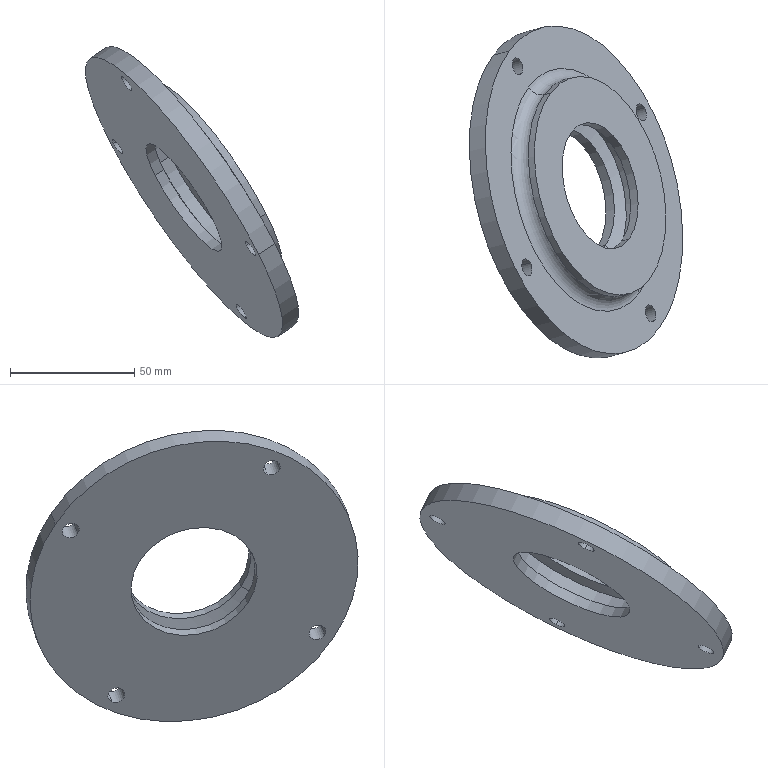Component | SolidWorks | InnerDustCover-1 | 1 solid | 27 faces | box 85.86 x 133.68 x 117.19 mm | volume 124699 mm3 | cylinder 18 | cone 4 | plane 3 | torus 2 | commonest cylinder face diameters 7 x8 52 x4 64 x2 90 x2 135 x2
STEP:
#1=CARTESIAN_POINT('',(-14.667,-7.905,-14.02));
#2=VERTEX_POINT('',#1);
#3=CARTESIAN_POINT('',(-16.423,-4.646,-12.677));
#4=VERTEX_POINT('',#3);
#5=CARTESIAN_POINT('',(-15.545,-6.275,-13.349));
#6=DIRECTION('',(-0.8088,-0.2094,-0.5495));
#7=DIRECTION('',(-0.4459,0.8276,0.341));
#8=AXIS2_PLACEMENT_3D('',#5,#6,#7);
#9=CIRCLE('',#8,1.969);
#10=EDGE_CURVE('',#2,#4,#9,.T.);
#11=ORIENTED_EDGE('',*,*,#10,.F.);
#12=CARTESIAN_POINT('',(-14.596,-7.7,-13.844));
#13=VERTEX_POINT('',#12);
#14=CARTESIAN_POINT('',(-14.508,-7.863,-13.912));
#15=DIRECTION('',(0.3834,0.5208,-0.7628));
#16=DIRECTION('',(0.,0.8259,0.5639));
#17=AXIS2_PLACEMENT_3D('',#14,#15,#16);
#18=CIRCLE('',#17,0.1969);
#19=EDGE_CURVE('',#2,#13,#18,.T.);
#20=ORIENTED_EDGE('',*,*,#19,.T.);
#21=CARTESIAN_POINT('',(-16.176,-4.768,-12.636));
#22=VERTEX_POINT('',#21);
#23=CARTESIAN_POINT('',(-15.386,-6.234,-13.24));
#24=DIRECTION('',(0.8088,0.2094,0.5495));
#25=DIRECTION('',(-0.4459,0.8276,0.341));
#26=AXIS2_PLACEMENT_3D('',#23,#24,#25);
#27=CIRCLE('',#26,1.772);
#28=EDGE_CURVE('',#22,#13,#27,.T.);
#29=ORIENTED_EDGE('',*,*,#28,.F.);
#30=CARTESIAN_POINT('',(-16.263,-4.605,-12.569));
#31=DIRECTION('',(-0.3834,-0.5208,0.7628));
#32=DIRECTION('',(0.,-0.8259,-0.5639));
#33=AXIS2_PLACEMENT_3D('',#30,#31,#32);
#34=CIRCLE('',#33,0.1969);
#35=EDGE_CURVE('',#4,#22,#34,.T.);
#36=ORIENTED_EDGE('',*,*,#35,.F.);
#37=EDGE_LOOP('',(#11,#20,#29,#36));
#38=FACE_OUTER_BOUND('',#37,.T.);
#39=CARTESIAN_POINT('',(-15.386,-6.234,-13.24));
#40=DIRECTION('',(-0.8088,-0.2094,-0.5495));
#41=DIRECTION('',(-0.4459,0.8276,0.341));
#42=AXIS2_PLACEMENT_3D('',#39,#40,#41);
#43=TOROIDAL_SURFACE('',#42,1.969,0.1969);
#44=ADVANCED_FACE('',(#38),#43,.F.);
#45=CARTESIAN_POINT('',(-14.841,-5.039,-15.429));
#46=VERTEX_POINT('',#45);
#47=CARTESIAN_POINT('',(-14.947,-5.183,-15.218));
#48=VERTEX_POINT('',#47);
#49=CARTESIAN_POINT('',(-14.894,-5.111,-15.323));
#50=DIRECTION('',(0.8088,0.2094,0.5495));
#51=DIRECTION('',(-0.3834,-0.5208,0.7628));
#52=AXIS2_PLACEMENT_3D('',#49,#50,#51);
#53=CIRCLE('',#52,0.1378);
#54=EDGE_CURVE('',#46,#48,#53,.T.);
#55=ORIENTED_EDGE('',*,*,#54,.F.);
#56=CARTESIAN_POINT('',(-14.587,-4.973,-15.255));
#57=VERTEX_POINT('',#56);
#58=CARTESIAN_POINT('',(-15.287,-5.155,-15.731));
#59=DIRECTION('',(0.8088,0.2094,0.5495));
#60=VECTOR('',#59,39.37);
#61=LINE('',#58,#60);
#62=EDGE_CURVE('',#46,#57,#61,.T.);
#63=ORIENTED_EDGE('',*,*,#62,.T.);
#64=CARTESIAN_POINT('',(-14.692,-5.117,-15.045));
#65=VERTEX_POINT('',#64);
#66=CARTESIAN_POINT('',(-14.639,-5.045,-15.15));
#67=DIRECTION('',(-0.8088,-0.2094,-0.5495));
#68=DIRECTION('',(0.3834,0.5208,-0.7628));
#69=AXIS2_PLACEMENT_3D('',#66,#67,#68);
#70=CIRCLE('',#69,0.1378);
#71=EDGE_CURVE('',#65,#57,#70,.T.);
#72=ORIENTED_EDGE('',*,*,#71,.F.);
#73=CARTESIAN_POINT('',(-15.393,-5.298,-15.521));
#74=DIRECTION('',(0.8088,0.2094,0.5495));
#75=VECTOR('',#74,39.37);
#76=LINE('',#73,#75);
#77=EDGE_CURVE('',#48,#65,#76,.T.);
#78=ORIENTED_EDGE('',*,*,#77,.F.);
#79=EDGE_LOOP('',(#55,#63,#72,#78));
#80=FACE_OUTER_BOUND('',#79,.T.);
#81=CARTESIAN_POINT('',(-15.34,-5.227,-15.626));
#82=DIRECTION('',(0.8088,0.2094,0.5495));
#83=DIRECTION('',(-0.3834,-0.5208,0.7628));
#84=AXIS2_PLACEMENT_3D('',#81,#82,#83);
#85=CYLINDRICAL_SURFACE('',#84,0.1378);
#86=ADVANCED_FACE('',(#80),#85,.F.);
#87=CARTESIAN_POINT('',(-14.685,-8.41,-14.374));
#88=VERTEX_POINT('',#87);
#89=CARTESIAN_POINT('',(-14.808,-8.182,-14.28));
#90=VERTEX_POINT('',#89);
#91=CARTESIAN_POINT('',(-14.746,-8.296,-14.327));
#92=DIRECTION('',(0.8088,0.2094,0.5495));
#93=DIRECTION('',(-0.4459,0.8276,0.341));
#94=AXIS2_PLACEMENT_3D('',#91,#92,#93);
#95=CIRCLE('',#94,0.1378);
#96=EDGE_CURVE('',#88,#90,#95,.T.);
#97=ORIENTED_EDGE('',*,*,#96,.F.);
#98=CARTESIAN_POINT('',(-14.43,-8.344,-14.201));
#99=VERTEX_POINT('',#98);
#100=CARTESIAN_POINT('',(-15.131,-8.526,-14.677));
#101=DIRECTION('',(0.8088,0.2094,0.5495));
#102=VECTOR('',#101,39.37);
#103=LINE('',#100,#102);
#104=EDGE_CURVE('',#88,#99,#103,.T.);
#105=ORIENTED_EDGE('',*,*,#104,.T.);
#106=CARTESIAN_POINT('',(-14.553,-8.116,-14.107));
#107=VERTEX_POINT('',#106);
#108=CARTESIAN_POINT('',(-14.492,-8.23,-14.154));
#109=DIRECTION('',(-0.8088,-0.2094,-0.5495));
#110=DIRECTION('',(0.4459,-0.8276,-0.341));
#111=AXIS2_PLACEMENT_3D('',#108,#109,#110);
#112=CIRCLE('',#111,0.1378);
#113=EDGE_CURVE('',#107,#99,#112,.T.);
#114=ORIENTED_EDGE('',*,*,#113,.F.);
#115=CARTESIAN_POINT('',(-15.254,-8.298,-14.583));
#116=DIRECTION('',(0.8088,0.2094,0.5495));
#117=VECTOR('',#116,39.37);
#118=LINE('',#115,#117);
#119=EDGE_CURVE('',#90,#107,#118,.T.);
#120=ORIENTED_EDGE('',*,*,#119,.F.);
#121=EDGE_LOOP('',(#97,#105,#114,#120));
#122=FACE_OUTER_BOUND('',#121,.T.);
#123=CARTESIAN_POINT('',(-15.192,-8.412,-14.63));
#124=DIRECTION('',(0.8088,0.2094,0.5495));
#125=DIRECTION('',(-0.4459,0.8276,0.341));
#126=AXIS2_PLACEMENT_3D('',#123,#124,#125);
#127=CYLINDRICAL_SURFACE('',#126,0.1378);
#128=ADVANCED_FACE('',(#122),#127,.F.);
#129=CARTESIAN_POINT('',(-16.758,-7.643,-11.615));
#130=VERTEX_POINT('',#129);
#131=CARTESIAN_POINT('',(-16.652,-7.5,-11.825));
#132=VERTEX_POINT('',#131);
#133=CARTESIAN_POINT('',(-16.705,-7.572,-11.72));
#134=DIRECTION('',(0.8088,0.2094,0.5495));
#135=DIRECTION('',(0.3834,0.5208,-0.7628));
#136=AXIS2_PLACEMENT_3D('',#133,#134,#135);
#137=CIRCLE('',#136,0.1378);
#138=EDGE_CURVE('',#130,#132,#137,.T.);
#139=ORIENTED_EDGE('',*,*,#138,.F.);
#140=CARTESIAN_POINT('',(-16.503,-7.577,-11.442));
#141=VERTEX_POINT('',#140);
#142=CARTESIAN_POINT('',(-17.204,-7.759,-11.918));
#143=DIRECTION('',(0.8088,0.2094,0.5495));
#144=VECTOR('',#143,39.37);
#145=LINE('',#142,#144);
#146=EDGE_CURVE('',#130,#141,#145,.T.);
#147=ORIENTED_EDGE('',*,*,#146,.T.);
#148=CARTESIAN_POINT('',(-16.398,-7.434,-11.652));
#149=VERTEX_POINT('',#148);
#150=CARTESIAN_POINT('',(-16.45,-7.506,-11.547));
#151=DIRECTION('',(-0.8088,-0.2094,-0.5495));
#152=DIRECTION('',(-0.3834,-0.5208,0.7628));
#153=AXIS2_PLACEMENT_3D('',#150,#151,#152);
#154=CIRCLE('',#153,0.1378);
#155=EDGE_CURVE('',#149,#141,#154,.T.);
#156=ORIENTED_EDGE('',*,*,#155,.F.);
#157=CARTESIAN_POINT('',(-17.098,-7.615,-12.128));
#158=DIRECTION('',(0.8088,0.2094,0.5495));
#159=VECTOR('',#158,39.37);
#160=LINE('',#157,#159);
#161=EDGE_CURVE('',#132,#149,#160,.T.);
#162=ORIENTED_EDGE('',*,*,#161,.F.);
#163=EDGE_LOOP('',(#139,#147,#156,#162));
#164=FACE_OUTER_BOUND('',#163,.T.);
#165=CARTESIAN_POINT('',(-17.151,-7.687,-12.023));
#166=DIRECTION('',(0.8088,0.2094,0.5495));
#167=DIRECTION('',(0.3834,0.5208,-0.7628));
#168=AXIS2_PLACEMENT_3D('',#165,#166,#167);
#169=CYLINDRICAL_SURFACE('',#168,0.1378);
#170=ADVANCED_FACE('',(#164),#169,.F.);
#171=CARTESIAN_POINT('',(-16.914,-4.272,-12.669));
#172=VERTEX_POINT('',#171);
#173=CARTESIAN_POINT('',(-16.792,-4.5,-12.763));
#174=VERTEX_POINT('',#173);
#175=CARTESIAN_POINT('',(-16.853,-4.386,-12.716));
#176=DIRECTION('',(0.8088,0.2094,0.5495));
#177=DIRECTION('',(0.4459,-0.8276,-0.341));
#178=AXIS2_PLACEMENT_3D('',#175,#176,#177);
#179=CIRCLE('',#178,0.1378);
#180=EDGE_CURVE('',#172,#174,#179,.T.);
#181=ORIENTED_EDGE('',*,*,#180,.F.);
#182=CARTESIAN_POINT('',(-16.66,-4.206,-12.496));
#183=VERTEX_POINT('',#182);
#184=CARTESIAN_POINT('',(-17.36,-4.388,-12.972));
#185=DIRECTION('',(0.8088,0.2094,0.5495));
#186=VECTOR('',#185,39.37);
#187=LINE('',#184,#186);
#188=EDGE_CURVE('',#172,#183,#187,.T.);
#189=ORIENTED_EDGE('',*,*,#188,.T.);
#190=CARTESIAN_POINT('',(-16.537,-4.434,-12.59));
#191=VERTEX_POINT('',#190);
#192=CARTESIAN_POINT('',(-16.598,-4.32,-12.543));
#193=DIRECTION('',(-0.8088,-0.2094,-0.5495));
#194=DIRECTION('',(-0.4459,0.8276,0.341));
#195=AXIS2_PLACEMENT_3D('',#192,#193,#194);
#196=CIRCLE('',#195,0.1378);
#197=EDGE_CURVE('',#191,#183,#196,.T.);
#198=ORIENTED_EDGE('',*,*,#197,.F.);
#199=CARTESIAN_POINT('',(-17.237,-4.616,-13.066));
#200=DIRECTION('',(0.8088,0.2094,0.5495));
#201=VECTOR('',#200,39.37);
#202=LINE('',#199,#201);
#203=EDGE_CURVE('',#174,#191,#202,.T.);
#204=ORIENTED_EDGE('',*,*,#203,.F.);
#205=EDGE_LOOP('',(#181,#189,#198,#204));
#206=FACE_OUTER_BOUND('',#205,.T.);
#207=CARTESIAN_POINT('',(-17.299,-4.502,-13.019));
#208=DIRECTION('',(0.8088,0.2094,0.5495));
#209=DIRECTION('',(0.4459,-0.8276,-0.341));
#210=AXIS2_PLACEMENT_3D('',#207,#208,#209);
#211=CYLINDRICAL_SURFACE('',#210,0.1378);
#212=ADVANCED_FACE('',(#206),#211,.F.);
#213=CARTESIAN_POINT('',(-15.208,-7.153,-13.779));
#214=VERTEX_POINT('',#213);
#215=CARTESIAN_POINT('',(-16.121,-5.459,-13.081));
#216=VERTEX_POINT('',#215);
#217=CARTESIAN_POINT('',(-15.664,-6.306,-13.43));
#218=DIRECTION('',(-0.8088,-0.2094,-0.5495));
#219=DIRECTION('',(-0.4459,0.8276,0.341));
#220=AXIS2_PLACEMENT_3D('',#217,#218,#219);
#221=CIRCLE('',#220,1.024);
#222=EDGE_CURVE('',#214,#216,#221,.T.);
#223=ORIENTED_EDGE('',*,*,#222,.T.);
#224=CARTESIAN_POINT('',(-16.178,-5.251,-12.968));
#225=VERTEX_POINT('',#224);
#226=CARTESIAN_POINT('',(-16.121,-5.459,-13.081));
#227=DIRECTION('',(-0.2364,0.8537,0.464));
#228=VECTOR('',#227,39.37);
#229=LINE('',#226,#228);
#230=EDGE_CURVE('',#216,#225,#229,.T.);
#231=ORIENTED_EDGE('',*,*,#230,.T.);
#232=CARTESIAN_POINT('',(-15.055,-7.337,-13.827));
#233=VERTEX_POINT('',#232);
#234=CARTESIAN_POINT('',(-15.617,-6.294,-13.397));
#235=DIRECTION('',(-0.8088,-0.2094,-0.5495));
#236=DIRECTION('',(-0.4459,0.8276,0.341));
#237=AXIS2_PLACEMENT_3D('',#234,#235,#236);
#238=CIRCLE('',#237,1.26);
#239=EDGE_CURVE('',#233,#225,#238,.T.);
#240=ORIENTED_EDGE('',*,*,#239,.F.);
#241=CARTESIAN_POINT('',(-15.208,-7.153,-13.779));
#242=DIRECTION('',(0.6288,-0.7521,-0.1975));
#243=VECTOR('',#242,39.37);
#244=LINE('',#241,#243);
#245=EDGE_CURVE('',#214,#233,#244,.T.);
#246=ORIENTED_EDGE('',*,*,#245,.F.);
#247=EDGE_LOOP('',(#223,#231,#240,#246));
#248=FACE_OUTER_BOUND('',#247,.T.);
#249=CARTESIAN_POINT('',(-15.664,-6.306,-13.43));
#250=DIRECTION('',(0.8088,0.2094,0.5495));
#251=DIRECTION('',(0.4459,-0.8276,-0.341));
#252=AXIS2_PLACEMENT_3D('',#249,#250,#251);
#253=CONICAL_SURFACE('',#252,1.024,1.326);
#254=ADVANCED_FACE('',(#248),#253,.F.);
#255=CARTESIAN_POINT('',(-14.896,-7.295,-13.719));
#256=VERTEX_POINT('',#255);
#257=CARTESIAN_POINT('',(-16.019,-5.21,-12.859));
#258=VERTEX_POINT('',#257);
#259=CARTESIAN_POINT('',(-15.457,-6.253,-13.289));
#260=DIRECTION('',(-0.8088,-0.2094,-0.5495));
#261=DIRECTION('',(-0.4459,0.8276,0.341));
#262=AXIS2_PLACEMENT_3D('',#259,#260,#261);
#263=CIRCLE('',#262,1.26);
#264=EDGE_CURVE('',#256,#258,#263,.T.);
#265=ORIENTED_EDGE('',*,*,#264,.F.);
#266=CARTESIAN_POINT('',(-15.238,-7.384,-13.951));
#267=DIRECTION('',(-0.8088,-0.2094,-0.5495));
#268=VECTOR('',#267,39.37);
#269=LINE('',#266,#268);
#270=EDGE_CURVE('',#256,#233,#269,.T.);
#271=ORIENTED_EDGE('',*,*,#270,.T.);
#272=ORIENTED_EDGE('',*,*,#239,.T.);
#273=CARTESIAN_POINT('',(-16.361,-5.299,-13.092));
#274=DIRECTION('',(-0.8088,-0.2094,-0.5495));
#275=VECTOR('',#274,39.37);
#276=LINE('',#273,#275);
#277=EDGE_CURVE('',#258,#225,#276,.T.);
#278=ORIENTED_EDGE('',*,*,#277,.F.);
#279=EDGE_LOOP('',(#265,#271,#272,#278));
#280=FACE_OUTER_BOUND('',#279,.T.);
#281=CARTESIAN_POINT('',(-15.8,-6.341,-13.522));
#282=DIRECTION('',(-0.8088,-0.2094,-0.5495));
#283=DIRECTION('',(-0.4459,0.8276,0.341));
#284=AXIS2_PLACEMENT_3D('',#281,#282,#283);
#285=CYLINDRICAL_SURFACE('',#284,1.26);
#286=ADVANCED_FACE('',(#280),#285,.F.);
#287=CARTESIAN_POINT('',(-14.953,-7.087,-13.606));
#288=VERTEX_POINT('',#287);
#289=CARTESIAN_POINT('',(-15.866,-5.393,-12.908));
#290=VERTEX_POINT('',#289);
#291=CARTESIAN_POINT('',(-15.41,-6.24,-13.257));
#292=DIRECTION('',(-0.8088,-0.2094,-0.5495));
#293=DIRECTION('',(-0.4459,0.8276,0.341));
#294=AXIS2_PLACEMENT_3D('',#291,#292,#293);
#295=CIRCLE('',#294,1.024);
#296=EDGE_CURVE('',#288,#290,#295,.T.);
#297=ORIENTED_EDGE('',*,*,#296,.F.);
#298=CARTESIAN_POINT('',(-14.896,-7.295,-13.719));
#299=DIRECTION('',(0.2364,-0.8537,-0.464));
#300=VECTOR('',#299,39.37);
#301=LINE('',#298,#300);
#302=EDGE_CURVE('',#288,#256,#301,.T.);
#303=ORIENTED_EDGE('',*,*,#302,.T.);
#304=ORIENTED_EDGE('',*,*,#264,.T.);
#305=CARTESIAN_POINT('',(-16.019,-5.21,-12.859));
#306=DIRECTION('',(-0.6288,0.7521,0.1975));
#307=VECTOR('',#306,39.37);
#308=LINE('',#305,#307);
#309=EDGE_CURVE('',#290,#258,#308,.T.);
#310=ORIENTED_EDGE('',*,*,#309,.F.);
#311=EDGE_LOOP('',(#297,#303,#304,#310));
#312=FACE_OUTER_BOUND('',#311,.T.);
#313=CARTESIAN_POINT('',(-15.457,-6.253,-13.289));
#314=DIRECTION('',(-0.8088,-0.2094,-0.5495));
#315=DIRECTION('',(-0.4459,0.8276,0.341));
#316=AXIS2_PLACEMENT_3D('',#313,#314,#315);
#317=CONICAL_SURFACE('',#316,1.26,1.326);
#318=ADVANCED_FACE('',(#312),#317,.F.);
#319=CARTESIAN_POINT('',(-14.834,-7.057,-13.524));
#320=VERTEX_POINT('',#319);
#321=CARTESIAN_POINT('',(-15.747,-5.362,-12.826));
#322=VERTEX_POINT('',#321);
#323=CARTESIAN_POINT('',(-15.29,-6.209,-13.175));
#324=DIRECTION('',(-0.8088,-0.2094,-0.5495));
#325=DIRECTION('',(-0.4459,0.8276,0.341));
#326=AXIS2_PLACEMENT_3D('',#323,#324,#325);
#327=CIRCLE('',#326,1.024);
#328=EDGE_CURVE('',#320,#322,#327,.T.);
#329=ORIENTED_EDGE('',*,*,#328,.F.);
#330=CARTESIAN_POINT('',(-15.343,-7.188,-13.871));
#331=DIRECTION('',(-0.8088,-0.2094,-0.5495));
#332=VECTOR('',#331,39.37);
#333=LINE('',#330,#332);
#334=EDGE_CURVE('',#320,#288,#333,.T.);
#335=ORIENTED_EDGE('',*,*,#334,.T.);
#336=ORIENTED_EDGE('',*,*,#296,.T.);
#337=CARTESIAN_POINT('',(-16.256,-5.494,-13.173));
#338=DIRECTION('',(-0.8088,-0.2094,-0.5495));
#339=VECTOR('',#338,39.37);
#340=LINE('',#337,#339);
#341=EDGE_CURVE('',#322,#290,#340,.T.);
#342=ORIENTED_EDGE('',*,*,#341,.F.);
#343=EDGE_LOOP('',(#329,#335,#336,#342));
#344=FACE_OUTER_BOUND('',#343,.T.);
#345=CARTESIAN_POINT('',(-15.8,-6.341,-13.522));
#346=DIRECTION('',(-0.8088,-0.2094,-0.5495));
#347=DIRECTION('',(-0.4459,0.8276,0.341));
#348=AXIS2_PLACEMENT_3D('',#345,#346,#347);
#349=CYLINDRICAL_SURFACE('',#348,1.024);
#350=ADVANCED_FACE('',(#344),#349,.F.);
#351=CARTESIAN_POINT('',(-16.08,-4.743,-12.571));
#352=VERTEX_POINT('',#351);
#353=CARTESIAN_POINT('',(-14.5,-7.676,-13.78));
#354=VERTEX_POINT('',#353);
#355=CARTESIAN_POINT('',(-15.29,-6.209,-13.175));
#356=DIRECTION('',(-0.8088,-0.2094,-0.5495));
#357=DIRECTION('',(-0.4459,0.8276,0.341));
#358=AXIS2_PLACEMENT_3D('',#355,#356,#357);
#359=CIRCLE('',#358,1.772);
#360=EDGE_CURVE('',#352,#354,#359,.T.);
#361=ORIENTED_EDGE('',*,*,#360,.T.);
#362=CARTESIAN_POINT('',(-15.01,-7.808,-14.126));
#363=DIRECTION('',(-0.8088,-0.2094,-0.5495));
#364=VECTOR('',#363,39.37);
#365=LINE('',#362,#364);
#366=EDGE_CURVE('',#354,#13,#365,.T.);
#367=ORIENTED_EDGE('',*,*,#366,.T.);
#368=CARTESIAN_POINT('',(-15.386,-6.234,-13.24));
#369=DIRECTION('',(0.8088,0.2094,0.5495));
#370=DIRECTION('',(-0.4459,0.8276,0.341));
#371=AXIS2_PLACEMENT_3D('',#368,#369,#370);
#372=CIRCLE('',#371,1.772);
#373=EDGE_CURVE('',#13,#22,#372,.T.);
#374=ORIENTED_EDGE('',*,*,#373,.T.);
#375=CARTESIAN_POINT('',(-16.59,-4.875,-12.918));
#376=DIRECTION('',(-0.8088,-0.2094,-0.5495));
#377=VECTOR('',#376,39.37);
#378=LINE('',#375,#377);
#379=EDGE_CURVE('',#352,#22,#378,.T.);
#380=ORIENTED_EDGE('',*,*,#379,.F.);
#381=EDGE_LOOP('',(#361,#367,#374,#380));
#382=FACE_OUTER_BOUND('',#381,.T.);
#383=CARTESIAN_POINT('',(-15.8,-6.341,-13.522));
#384=DIRECTION('',(-0.8088,-0.2094,-0.5495));
#385=DIRECTION('',(-0.4459,0.8276,0.341));
#386=AXIS2_PLACEMENT_3D('',#383,#384,#385);
#387=CYLINDRICAL_SURFACE('',#386,1.772);
#388=ADVANCED_FACE('',(#382),#387,.T.);
#389=CARTESIAN_POINT('',(-16.73,-4.076,-12.442));
#390=VERTEX_POINT('',#389);
#391=CARTESIAN_POINT('',(-14.36,-8.475,-14.255));
#392=VERTEX_POINT('',#391);
#393=CARTESIAN_POINT('',(-15.545,-6.275,-13.349));
#394=DIRECTION('',(-0.8088,-0.2094,-0.5495));
#395=DIRECTION('',(-0.4459,0.8276,0.341));
#396=AXIS2_PLACEMENT_3D('',#393,#394,#395);
#397=CIRCLE('',#396,2.657);
#398=EDGE_CURVE('',#390,#392,#397,.T.);
#399=ORIENTED_EDGE('',*,*,#398,.T.);
#400=CARTESIAN_POINT('',(-14.615,-8.541,-14.428));
#401=VERTEX_POINT('',#400);
#402=CARTESIAN_POINT('',(-14.615,-8.541,-14.428));
#403=DIRECTION('',(-0.8088,-0.2094,-0.5495));
#404=VECTOR('',#403,39.37);
#405=LINE('',#402,#404);
#406=EDGE_CURVE('',#392,#401,#405,.T.);
#407=ORIENTED_EDGE('',*,*,#406,.T.);
#408=CARTESIAN_POINT('',(-16.985,-4.142,-12.615));
#409=VERTEX_POINT('',#408);
#410=CARTESIAN_POINT('',(-15.8,-6.341,-13.522));
#411=DIRECTION('',(-0.8088,-0.2094,-0.5495));
#412=DIRECTION('',(-0.4459,0.8276,0.341));
#413=AXIS2_PLACEMENT_3D('',#410,#411,#412);
#414=CIRCLE('',#413,2.657);
#415=EDGE_CURVE('',#409,#401,#414,.T.);
#416=ORIENTED_EDGE('',*,*,#415,.F.);
#417=CARTESIAN_POINT('',(-16.985,-4.142,-12.615));
#418=DIRECTION('',(-0.8088,-0.2094,-0.5495));
#419=VECTOR('',#418,39.37);
#420=LINE('',#417,#419);
#421=EDGE_CURVE('',#390,#409,#420,.T.);
#422=ORIENTED_EDGE('',*,*,#421,.F.);
#423=EDGE_LOOP('',(#399,#407,#416,#422));
#424=FACE_OUTER_BOUND('',#423,.T.);
#425=CARTESIAN_POINT('',(-15.8,-6.341,-13.522));
#426=DIRECTION('',(-0.8088,-0.2094,-0.5495));
#427=DIRECTION('',(-0.4459,0.8276,0.341));
#428=AXIS2_PLACEMENT_3D('',#425,#426,#427);
#429=CYLINDRICAL_SURFACE('',#428,2.657);
#430=ADVANCED_FACE('',(#424),#429,.T.);
#431=ORIENTED_EDGE('',*,*,#222,.F.);
#432=CARTESIAN_POINT('',(-15.343,-7.188,-13.871));
#433=VERTEX_POINT('',#432);
#434=CARTESIAN_POINT('',(-15.343,-7.188,-13.871));
#435=DIRECTION('',(-0.8088,-0.2094,-0.5495));
#436=VECTOR('',#435,39.37);
#437=LINE('',#434,#436);
#438=EDGE_CURVE('',#214,#433,#437,.T.);
#439=ORIENTED_EDGE('',*,*,#438,.T.);
#440=CARTESIAN_POINT('',(-16.256,-5.494,-13.173));
#441=VERTEX_POINT('',#440);
#442=CARTESIAN_POINT('',(-15.8,-6.341,-13.522));
#443=DIRECTION('',(-0.8088,-0.2094,-0.5495));
#444=DIRECTION('',(-0.4459,0.8276,0.341));
#445=AXIS2_PLACEMENT_3D('',#442,#443,#444);
#446=CIRCLE('',#445,1.024);
#447=EDGE_CURVE('',#433,#441,#446,.T.);
#448=ORIENTED_EDGE('',*,*,#447,.T.);
#449=CARTESIAN_POINT('',(-16.256,-5.494,-13.173));
#450=DIRECTION('',(-0.8088,-0.2094,-0.5495));
#451=VECTOR('',#450,39.37);
#452=LINE('',#449,#451);
#453=EDGE_CURVE('',#216,#441,#452,.T.);
#454=ORIENTED_EDGE('',*,*,#453,.F.);
#455=EDGE_LOOP('',(#431,#439,#448,#454));
#456=FACE_OUTER_BOUND('',#455,.T.);
#457=CARTESIAN_POINT('',(-15.8,-6.341,-13.522));
#458=DIRECTION('',(-0.8088,-0.2094,-0.5495));
#459=DIRECTION('',(-0.4459,0.8276,0.341));
#460=AXIS2_PLACEMENT_3D('',#457,#458,#459);
#461=CYLINDRICAL_SURFACE('',#460,1.024);
#462=ADVANCED_FACE('',(#456),#461,.F.);
#463=ORIENTED_EDGE('',*,*,#438,.F.);
#464=CARTESIAN_POINT('',(-15.664,-6.306,-13.43));
#465=DIRECTION('',(-0.8088,-0.2094,-0.5495));
#466=DIRECTION('',(-0.4459,0.8276,0.341));
#467=AXIS2_PLACEMENT_3D('',#464,#465,#466);
#468=CIRCLE('',#467,1.024);
#469=EDGE_CURVE('',#216,#214,#468,.T.);
#470=ORIENTED_EDGE('',*,*,#469,.F.);
#471=ORIENTED_EDGE('',*,*,#453,.T.);
#472=CARTESIAN_POINT('',(-15.8,-6.341,-13.522));
#473=DIRECTION('',(-0.8088,-0.2094,-0.5495));
#474=DIRECTION('',(-0.4459,0.8276,0.341));
#475=AXIS2_PLACEMENT_3D('',#472,#473,#474);
#476=CIRCLE('',#475,1.024);
#477=EDGE_CURVE('',#441,#433,#476,.T.);
#478=ORIENTED_EDGE('',*,*,#477,.T.);
#479=EDGE_LOOP('',(#463,#470,#471,#478));
#480=FACE_OUTER_BOUND('',#479,.T.);
#481=CARTESIAN_POINT('',(-15.8,-6.341,-13.522));
#482=DIRECTION('',(-0.8088,-0.2094,-0.5495));
#483=DIRECTION('',(-0.4459,0.8276,0.341));
#484=AXIS2_PLACEMENT_3D('',#481,#482,#483);
#485=CYLINDRICAL_SURFACE('',#484,1.024);
#486=ADVANCED_FACE('',(#480),#485,.F.);
#487=CARTESIAN_POINT('',(-14.894,-5.111,-15.323));
#488=DIRECTION('',(0.8088,0.2094,0.5495));
#489=DIRECTION('',(-0.3834,-0.5208,0.7628));
#490=AXIS2_PLACEMENT_3D('',#487,#488,#489);
#491=CIRCLE('',#490,0.1378);
#492=EDGE_CURVE('',#48,#46,#491,.T.);
#493=ORIENTED_EDGE('',*,*,#492,.T.);
#494=ORIENTED_EDGE('',*,*,#54,.T.);
#495=EDGE_LOOP('',(#493,#494));
#496=FACE_BOUND('',#495,.T.);
#497=CARTESIAN_POINT('',(-14.746,-8.296,-14.327));
#498=DIRECTION('',(0.8088,0.2094,0.5495));
#499=DIRECTION('',(-0.4459,0.8276,0.341));
#500=AXIS2_PLACEMENT_3D('',#497,#498,#499);
#501=CIRCLE('',#500,0.1378);
#502=EDGE_CURVE('',#90,#88,#501,.T.);
#503=ORIENTED_EDGE('',*,*,#502,.T.);
#504=ORIENTED_EDGE('',*,*,#96,.T.);
#505=EDGE_LOOP('',(#503,#504));
#506=FACE_BOUND('',#505,.T.);
#507=CARTESIAN_POINT('',(-16.705,-7.572,-11.72));
#508=DIRECTION('',(0.8088,0.2094,0.5495));
#509=DIRECTION('',(0.3834,0.5208,-0.7628));
#510=AXIS2_PLACEMENT_3D('',#507,#508,#509);
#511=CIRCLE('',#510,0.1378);
#512=EDGE_CURVE('',#132,#130,#511,.T.);
#513=ORIENTED_EDGE('',*,*,#512,.T.);
#514=ORIENTED_EDGE('',*,*,#138,.T.);
#515=EDGE_LOOP('',(#513,#514));
#516=FACE_BOUND('',#515,.T.);
#517=CARTESIAN_POINT('',(-16.853,-4.386,-12.716));
#518=DIRECTION('',(0.8088,0.2094,0.5495));
#519=DIRECTION('',(0.4459,-0.8276,-0.341));
#520=AXIS2_PLACEMENT_3D('',#517,#518,#519);
#521=CIRCLE('',#520,0.1378);
#522=EDGE_CURVE('',#174,#172,#521,.T.);
#523=ORIENTED_EDGE('',*,*,#522,.T.);
#524=ORIENTED_EDGE('',*,*,#180,.T.);
#525=EDGE_LOOP('',(#523,#524));
#526=FACE_BOUND('',#525,.T.);
#527=ORIENTED_EDGE('',*,*,#477,.F.);
#528=ORIENTED_EDGE('',*,*,#447,.F.);
#529=EDGE_LOOP('',(#527,#528));
#530=FACE_BOUND('',#529,.T.);
#531=ORIENTED_EDGE('',*,*,#415,.T.);
#532=CARTESIAN_POINT('',(-15.8,-6.341,-13.522));
#533=DIRECTION('',(-0.8088,-0.2094,-0.5495));
#534=DIRECTION('',(-0.4459,0.8276,0.341));
#535=AXIS2_PLACEMENT_3D('',#532,#533,#534);
#536=CIRCLE('',#535,2.657);
#537=EDGE_CURVE('',#401,#409,#536,.T.);
#538=ORIENTED_EDGE('',*,*,#537,.T.);
#539=EDGE_LOOP('',(#531,#538));
#540=FACE_OUTER_BOUND('',#539,.T.);
#541=CARTESIAN_POINT('',(-15.407,-5.808,-14.302));
#542=DIRECTION('',(0.8088,0.2094,0.5495));
#543=DIRECTION('',(0.4459,-0.8276,-0.341));
#544=AXIS2_PLACEMENT_3D('',#541,#542,#543);
#545=PLANE('',#544);
#546=ADVANCED_FACE('',(#496,#506,#516,#526,#530,#540),#545,.F.);
#547=ORIENTED_EDGE('',*,*,#406,.F.);
#548=CARTESIAN_POINT('',(-15.545,-6.275,-13.349));
#549=DIRECTION('',(-0.8088,-0.2094,-0.5495));
#550=DIRECTION('',(-0.4459,0.8276,0.341));
#551=AXIS2_PLACEMENT_3D('',#548,#549,#550);
#552=CIRCLE('',#551,2.657);
#553=EDGE_CURVE('',#392,#390,#552,.T.);
#554=ORIENTED_EDGE('',*,*,#553,.T.);
#555=ORIENTED_EDGE('',*,*,#421,.T.);
#556=ORIENTED_EDGE('',*,*,#537,.F.);
#557=EDGE_LOOP('',(#547,#554,#555,#556));
#558=FACE_OUTER_BOUND('',#557,.T.);
#559=CARTESIAN_POINT('',(-15.8,-6.341,-13.522));
#560=DIRECTION('',(-0.8088,-0.2094,-0.5495));
#561=DIRECTION('',(-0.4459,0.8276,0.341));
#562=AXIS2_PLACEMENT_3D('',#559,#560,#561);
#563=CYLINDRICAL_SURFACE('',#562,2.657);
#564=ADVANCED_FACE('',(#558),#563,.T.);
#565=CARTESIAN_POINT('',(-15.545,-6.275,-13.349));
#566=DIRECTION('',(-0.8088,-0.2094,-0.5495));
#567=DIRECTION('',(-0.4459,0.8276,0.341));
#568=AXIS2_PLACEMENT_3D('',#565,#566,#567);
#569=CIRCLE('',#568,1.969);
#570=EDGE_CURVE('',#4,#2,#569,.T.);
#571=ORIENTED_EDGE('',*,*,#570,.T.);
#572=ORIENTED_EDGE('',*,*,#10,.T.);
#573=EDGE_LOOP('',(#571,#572));
#574=FACE_BOUND('',#573,.T.);
#575=ORIENTED_EDGE('',*,*,#71,.T.);
#576=CARTESIAN_POINT('',(-14.639,-5.045,-15.15));
#577=DIRECTION('',(-0.8088,-0.2094,-0.5495));
#578=DIRECTION('',(0.3834,0.5208,-0.7628));
#579=AXIS2_PLACEMENT_3D('',#576,#577,#578);
#580=CIRCLE('',#579,0.1378);
#581=EDGE_CURVE('',#57,#65,#580,.T.);
#582=ORIENTED_EDGE('',*,*,#581,.T.);
#583=EDGE_LOOP('',(#575,#582));
#584=FACE_BOUND('',#583,.T.);
#585=ORIENTED_EDGE('',*,*,#113,.T.);
#586=CARTESIAN_POINT('',(-14.492,-8.23,-14.154));
#587=DIRECTION('',(-0.8088,-0.2094,-0.5495));
#588=DIRECTION('',(0.4459,-0.8276,-0.341));
#589=AXIS2_PLACEMENT_3D('',#586,#587,#588);
#590=CIRCLE('',#589,0.1378);
#591=EDGE_CURVE('',#99,#107,#590,.T.);
#592=ORIENTED_EDGE('',*,*,#591,.T.);
#593=EDGE_LOOP('',(#585,#592));
#594=FACE_BOUND('',#593,.T.);
#595=ORIENTED_EDGE('',*,*,#155,.T.);
#596=CARTESIAN_POINT('',(-16.45,-7.506,-11.547));
#597=DIRECTION('',(-0.8088,-0.2094,-0.5495));
#598=DIRECTION('',(-0.3834,-0.5208,0.7628));
#599=AXIS2_PLACEMENT_3D('',#596,#597,#598);
#600=CIRCLE('',#599,0.1378);
#601=EDGE_CURVE('',#141,#149,#600,.T.);
#602=ORIENTED_EDGE('',*,*,#601,.T.);
#603=EDGE_LOOP('',(#595,#602));
#604=FACE_BOUND('',#603,.T.);
#605=ORIENTED_EDGE('',*,*,#197,.T.);
#606=CARTESIAN_POINT('',(-16.598,-4.32,-12.543));
#607=DIRECTION('',(-0.8088,-0.2094,-0.5495));
#608=DIRECTION('',(-0.4459,0.8276,0.341));
#609=AXIS2_PLACEMENT_3D('',#606,#607,#608);
#610=CIRCLE('',#609,0.1378);
#611=EDGE_CURVE('',#183,#191,#610,.T.);
#612=ORIENTED_EDGE('',*,*,#611,.T.);
#613=EDGE_LOOP('',(#605,#612));
#614=FACE_BOUND('',#613,.T.);
#615=ORIENTED_EDGE('',*,*,#398,.F.);
#616=ORIENTED_EDGE('',*,*,#553,.F.);
#617=EDGE_LOOP('',(#615,#616));
#618=FACE_OUTER_BOUND('',#617,.T.);
#619=CARTESIAN_POINT('',(-14.526,-4.891,-15.376));
#620=DIRECTION('',(-0.8088,-0.2094,-0.5495));
#621=DIRECTION('',(-0.4459,0.8276,0.341));
#622=AXIS2_PLACEMENT_3D('',#619,#620,#621);
#623=PLANE('',#622);
#624=ADVANCED_FACE('',(#574,#584,#594,#604,#614,#618),#623,.F.);
#625=ORIENTED_EDGE('',*,*,#366,.F.);
#626=CARTESIAN_POINT('',(-15.29,-6.209,-13.175));
#627=DIRECTION('',(-0.8088,-0.2094,-0.5495));
#628=DIRECTION('',(-0.4459,0.8276,0.341));
#629=AXIS2_PLACEMENT_3D('',#626,#627,#628);
#630=CIRCLE('',#629,1.772);
#631=EDGE_CURVE('',#354,#352,#630,.T.);
#632=ORIENTED_EDGE('',*,*,#631,.T.);
#633=ORIENTED_EDGE('',*,*,#379,.T.);
#634=ORIENTED_EDGE('',*,*,#28,.T.);
#635=EDGE_LOOP('',(#625,#632,#633,#634));
#636=FACE_OUTER_BOUND('',#635,.T.);
#637=CARTESIAN_POINT('',(-15.8,-6.341,-13.522));
#638=DIRECTION('',(-0.8088,-0.2094,-0.5495));
#639=DIRECTION('',(-0.4459,0.8276,0.341));
#640=AXIS2_PLACEMENT_3D('',#637,#638,#639);
#641=CYLINDRICAL_SURFACE('',#640,1.772);
#642=ADVANCED_FACE('',(#636),#641,.T.);
#643=ORIENTED_EDGE('',*,*,#360,.F.);
#644=ORIENTED_EDGE('',*,*,#631,.F.);
#645=EDGE_LOOP('',(#643,#644));
#646=FACE_OUTER_BOUND('',#645,.T.);
#647=CARTESIAN_POINT('',(-15.29,-6.209,-13.175));
#648=DIRECTION('',(-0.8088,-0.2094,-0.5495));
#649=DIRECTION('',(-0.4459,0.8276,0.341));
#650=AXIS2_PLACEMENT_3D('',#647,#648,#649);
#651=CIRCLE('',#650,1.024);
#652=EDGE_CURVE('',#322,#320,#651,.T.);
#653=ORIENTED_EDGE('',*,*,#652,.T.);
#654=ORIENTED_EDGE('',*,*,#328,.T.);
#655=EDGE_LOOP('',(#653,#654));
#656=FACE_BOUND('',#655,.T.);
#657=CARTESIAN_POINT('',(-14.611,-5.287,-14.527));
#658=DIRECTION('',(-0.8088,-0.2094,-0.5495));
#659=DIRECTION('',(-0.4459,0.8276,0.341));
#660=AXIS2_PLACEMENT_3D('',#657,#658,#659);
#661=PLANE('',#660);
#662=ADVANCED_FACE('',(#646,#656),#661,.F.);
#663=ORIENTED_EDGE('',*,*,#334,.F.);
#664=ORIENTED_EDGE('',*,*,#652,.F.);
#665=ORIENTED_EDGE('',*,*,#341,.T.);
#666=CARTESIAN_POINT('',(-15.41,-6.24,-13.257));
#667=DIRECTION('',(-0.8088,-0.2094,-0.5495));
#668=DIRECTION('',(-0.4459,0.8276,0.341));
#669=AXIS2_PLACEMENT_3D('',#666,#667,#668);
#670=CIRCLE('',#669,1.024);
#671=EDGE_CURVE('',#290,#288,#670,.T.);
#672=ORIENTED_EDGE('',*,*,#671,.T.);
#673=EDGE_LOOP('',(#663,#664,#665,#672));
#674=FACE_OUTER_BOUND('',#673,.T.);
#675=CARTESIAN_POINT('',(-15.8,-6.341,-13.522));
#676=DIRECTION('',(-0.8088,-0.2094,-0.5495));
#677=DIRECTION('',(-0.4459,0.8276,0.341));
#678=AXIS2_PLACEMENT_3D('',#675,#676,#677);
#679=CYLINDRICAL_SURFACE('',#678,1.024);
#680=ADVANCED_FACE('',(#674),#679,.F.);
#681=ORIENTED_EDGE('',*,*,#302,.F.);
#682=ORIENTED_EDGE('',*,*,#671,.F.);
#683=ORIENTED_EDGE('',*,*,#309,.T.);
#684=CARTESIAN_POINT('',(-15.457,-6.253,-13.289));
#685=DIRECTION('',(-0.8088,-0.2094,-0.5495));
#686=DIRECTION('',(-0.4459,0.8276,0.341));
#687=AXIS2_PLACEMENT_3D('',#684,#685,#686);
#688=CIRCLE('',#687,1.26);
#689=EDGE_CURVE('',#258,#256,#688,.T.);
#690=ORIENTED_EDGE('',*,*,#689,.T.);
#691=EDGE_LOOP('',(#681,#682,#683,#690));
#692=FACE_OUTER_BOUND('',#691,.T.);
#693=CARTESIAN_POINT('',(-15.457,-6.253,-13.289));
#694=DIRECTION('',(-0.8088,-0.2094,-0.5495));
#695=DIRECTION('',(-0.4459,0.8276,0.341));
#696=AXIS2_PLACEMENT_3D('',#693,#694,#695);
#697=CONICAL_SURFACE('',#696,1.26,1.326);
#698=ADVANCED_FACE('',(#692),#697,.F.);
#699=ORIENTED_EDGE('',*,*,#270,.F.);
#700=ORIENTED_EDGE('',*,*,#689,.F.);
#701=ORIENTED_EDGE('',*,*,#277,.T.);
#702=CARTESIAN_POINT('',(-15.617,-6.294,-13.397));
#703=DIRECTION('',(-0.8088,-0.2094,-0.5495));
#704=DIRECTION('',(-0.4459,0.8276,0.341));
#705=AXIS2_PLACEMENT_3D('',#702,#703,#704);
#706=CIRCLE('',#705,1.26);
#707=EDGE_CURVE('',#225,#233,#706,.T.);
#708=ORIENTED_EDGE('',*,*,#707,.T.);
#709=EDGE_LOOP('',(#699,#700,#701,#708));
#710=FACE_OUTER_BOUND('',#709,.T.);
#711=CARTESIAN_POINT('',(-15.8,-6.341,-13.522));
#712=DIRECTION('',(-0.8088,-0.2094,-0.5495));
#713=DIRECTION('',(-0.4459,0.8276,0.341));
#714=AXIS2_PLACEMENT_3D('',#711,#712,#713);
#715=CYLINDRICAL_SURFACE('',#714,1.26);
#716=ADVANCED_FACE('',(#710),#715,.F.);
#717=ORIENTED_EDGE('',*,*,#230,.F.);
#718=ORIENTED_EDGE('',*,*,#469,.T.);
#719=ORIENTED_EDGE('',*,*,#245,.T.);
#720=ORIENTED_EDGE('',*,*,#707,.F.);
#721=EDGE_LOOP('',(#717,#718,#719,#720));
#722=FACE_OUTER_BOUND('',#721,.T.);
#723=CARTESIAN_POINT('',(-15.664,-6.306,-13.43));
#724=DIRECTION('',(0.8088,0.2094,0.5495));
#725=DIRECTION('',(0.4459,-0.8276,-0.341));
#726=AXIS2_PLACEMENT_3D('',#723,#724,#725);
#727=CONICAL_SURFACE('',#726,1.024,1.326);
#728=ADVANCED_FACE('',(#722),#727,.F.);
#729=ORIENTED_EDGE('',*,*,#188,.F.);
#730=ORIENTED_EDGE('',*,*,#522,.F.);
#731=ORIENTED_EDGE('',*,*,#203,.T.);
#732=ORIENTED_EDGE('',*,*,#611,.F.);
#733=EDGE_LOOP('',(#729,#730,#731,#732));
#734=FACE_OUTER_BOUND('',#733,.T.);
#735=CARTESIAN_POINT('',(-17.299,-4.502,-13.019));
#736=DIRECTION('',(0.8088,0.2094,0.5495));
#737=DIRECTION('',(0.4459,-0.8276,-0.341));
#738=AXIS2_PLACEMENT_3D('',#735,#736,#737);
#739=CYLINDRICAL_SURFACE('',#738,0.1378);
#740=ADVANCED_FACE('',(#734),#739,.F.);
#741=ORIENTED_EDGE('',*,*,#146,.F.);
#742=ORIENTED_EDGE('',*,*,#512,.F.);
#743=ORIENTED_EDGE('',*,*,#161,.T.);
#744=ORIENTED_EDGE('',*,*,#601,.F.);
#745=EDGE_LOOP('',(#741,#742,#743,#744));
#746=FACE_OUTER_BOUND('',#745,.T.);
#747=CARTESIAN_POINT('',(-17.151,-7.687,-12.023));
#748=DIRECTION('',(0.8088,0.2094,0.5495));
#749=DIRECTION('',(0.3834,0.5208,-0.7628));
#750=AXIS2_PLACEMENT_3D('',#747,#748,#749);
#751=CYLINDRICAL_SURFACE('',#750,0.1378);
#752=ADVANCED_FACE('',(#746),#751,.F.);
#753=ORIENTED_EDGE('',*,*,#104,.F.);
#754=ORIENTED_EDGE('',*,*,#502,.F.);
#755=ORIENTED_EDGE('',*,*,#119,.T.);
#756=ORIENTED_EDGE('',*,*,#591,.F.);
#757=EDGE_LOOP('',(#753,#754,#755,#756));
#758=FACE_OUTER_BOUND('',#757,.T.);
#759=CARTESIAN_POINT('',(-15.192,-8.412,-14.63));
#760=DIRECTION('',(0.8088,0.2094,0.5495));
#761=DIRECTION('',(-0.4459,0.8276,0.341));
#762=AXIS2_PLACEMENT_3D('',#759,#760,#761);
#763=CYLINDRICAL_SURFACE('',#762,0.1378);
#764=ADVANCED_FACE('',(#758),#763,.F.);
#765=ORIENTED_EDGE('',*,*,#62,.F.);
#766=ORIENTED_EDGE('',*,*,#492,.F.);
#767=ORIENTED_EDGE('',*,*,#77,.T.);
#768=ORIENTED_EDGE('',*,*,#581,.F.);
#769=EDGE_LOOP('',(#765,#766,#767,#768));
#770=FACE_OUTER_BOUND('',#769,.T.);
#771=CARTESIAN_POINT('',(-15.34,-5.227,-15.626));
#772=DIRECTION('',(0.8088,0.2094,0.5495));
#773=DIRECTION('',(-0.3834,-0.5208,0.7628));
#774=AXIS2_PLACEMENT_3D('',#771,#772,#773);
#775=CYLINDRICAL_SURFACE('',#774,0.1378);
#776=ADVANCED_FACE('',(#770),#775,.F.);
#777=ORIENTED_EDGE('',*,*,#19,.F.);
#778=ORIENTED_EDGE('',*,*,#570,.F.);
#779=ORIENTED_EDGE('',*,*,#35,.T.);
#780=ORIENTED_EDGE('',*,*,#373,.F.);
#781=EDGE_LOOP('',(#777,#778,#779,#780));
#782=FACE_OUTER_BOUND('',#781,.T.);
#783=CARTESIAN_POINT('',(-15.386,-6.234,-13.24));
#784=DIRECTION('',(-0.8088,-0.2094,-0.5495));
#785=DIRECTION('',(-0.4459,0.8276,0.341));
#786=AXIS2_PLACEMENT_3D('',#783,#784,#785);
#787=TOROIDAL_SURFACE('',#786,1.969,0.1969);
#788=ADVANCED_FACE('',(#782),#787,.F.);
#789=CLOSED_SHELL('',(#44,#86,#128,#170,#212,#254,#286,#318,#350,#388,#430,#462,#486,#546,#564,#624,#642,#662,#680,#698,#716,#728,#740,#752,#764,#776,#788));
#790=MANIFOLD_SOLID_BREP('',#789);
#791=CARTESIAN_POINT('',(0.,0.,0.));
#792=DIRECTION('',(0.,0.,1.));
#793=DIRECTION('',(1.,0.,0.));
#794=AXIS2_PLACEMENT_3D('',#791,#792,#793);
#795=(LENGTH_UNIT()NAMED_UNIT(*)SI_UNIT($,.METRE.));
#796=LENGTH_MEASURE_WITH_UNIT(LENGTH_MEASURE(0.0254),#795);
#797=DIMENSIONAL_EXPONENTS(1.,0.,0.,0.,0.,0.,0.);
#798=(CONVERSION_BASED_UNIT('',#796)LENGTH_UNIT()NAMED_UNIT(#797));
#799=UNCERTAINTY_MEASURE_WITH_UNIT(LENGTH_MEASURE(0.00001),#798,'','');
#800=(NAMED_UNIT(*)PLANE_ANGLE_UNIT()SI_UNIT($,.RADIAN.));
#801=(NAMED_UNIT(*)SI_UNIT($,.STERADIAN.)SOLID_ANGLE_UNIT());
#802=(GEOMETRIC_REPRESENTATION_CONTEXT(3)GLOBAL_UNCERTAINTY_ASSIGNED_CONTEXT((#799))GLOBAL_UNIT_ASSIGNED_CONTEXT((#798,#800,#801))REPRESENTATION_CONTEXT('',''));
#803=ADVANCED_BREP_SHAPE_REPRESENTATION('',(#790,#794),#802);
#804=COLOUR_RGB('',0.7922,0.8196,0.9333);
#805=FILL_AREA_STYLE_COLOUR('',#804);
#806=FILL_AREA_STYLE('',(#805));
#807=SURFACE_STYLE_FILL_AREA(#806);
#808=SURFACE_SIDE_STYLE('',(#807));
#809=SURFACE_STYLE_USAGE(.BOTH.,#808);
#810=PRESENTATION_STYLE_ASSIGNMENT((#809));
#811=STYLED_ITEM('',(#810),#790);
#812=(LENGTH_UNIT()NAMED_UNIT(*)SI_UNIT($,.METRE.));
#813=LENGTH_MEASURE_WITH_UNIT(LENGTH_MEASURE(0.0254),#812);
#814=DIMENSIONAL_EXPONENTS(1.,0.,0.,0.,0.,0.,0.);
#815=(CONVERSION_BASED_UNIT('',#813)LENGTH_UNIT()NAMED_UNIT(#814));
#816=UNCERTAINTY_MEASURE_WITH_UNIT(LENGTH_MEASURE(0.00001),#815,'','');
#817=(NAMED_UNIT(*)PLANE_ANGLE_UNIT()SI_UNIT($,.RADIAN.));
#818=(NAMED_UNIT(*)SI_UNIT($,.STERADIAN.)SOLID_ANGLE_UNIT());
#819=(GEOMETRIC_REPRESENTATION_CONTEXT(3)GLOBAL_UNCERTAINTY_ASSIGNED_CONTEXT((#816))GLOBAL_UNIT_ASSIGNED_CONTEXT((#815,#817,#818))REPRESENTATION_CONTEXT('',''));
#820=MECHANICAL_DESIGN_GEOMETRIC_PRESENTATION_REPRESENTATION('',(#811),#819);
#821=PRESENTATION_LAYER_ASSIGNMENT('','',(#811));